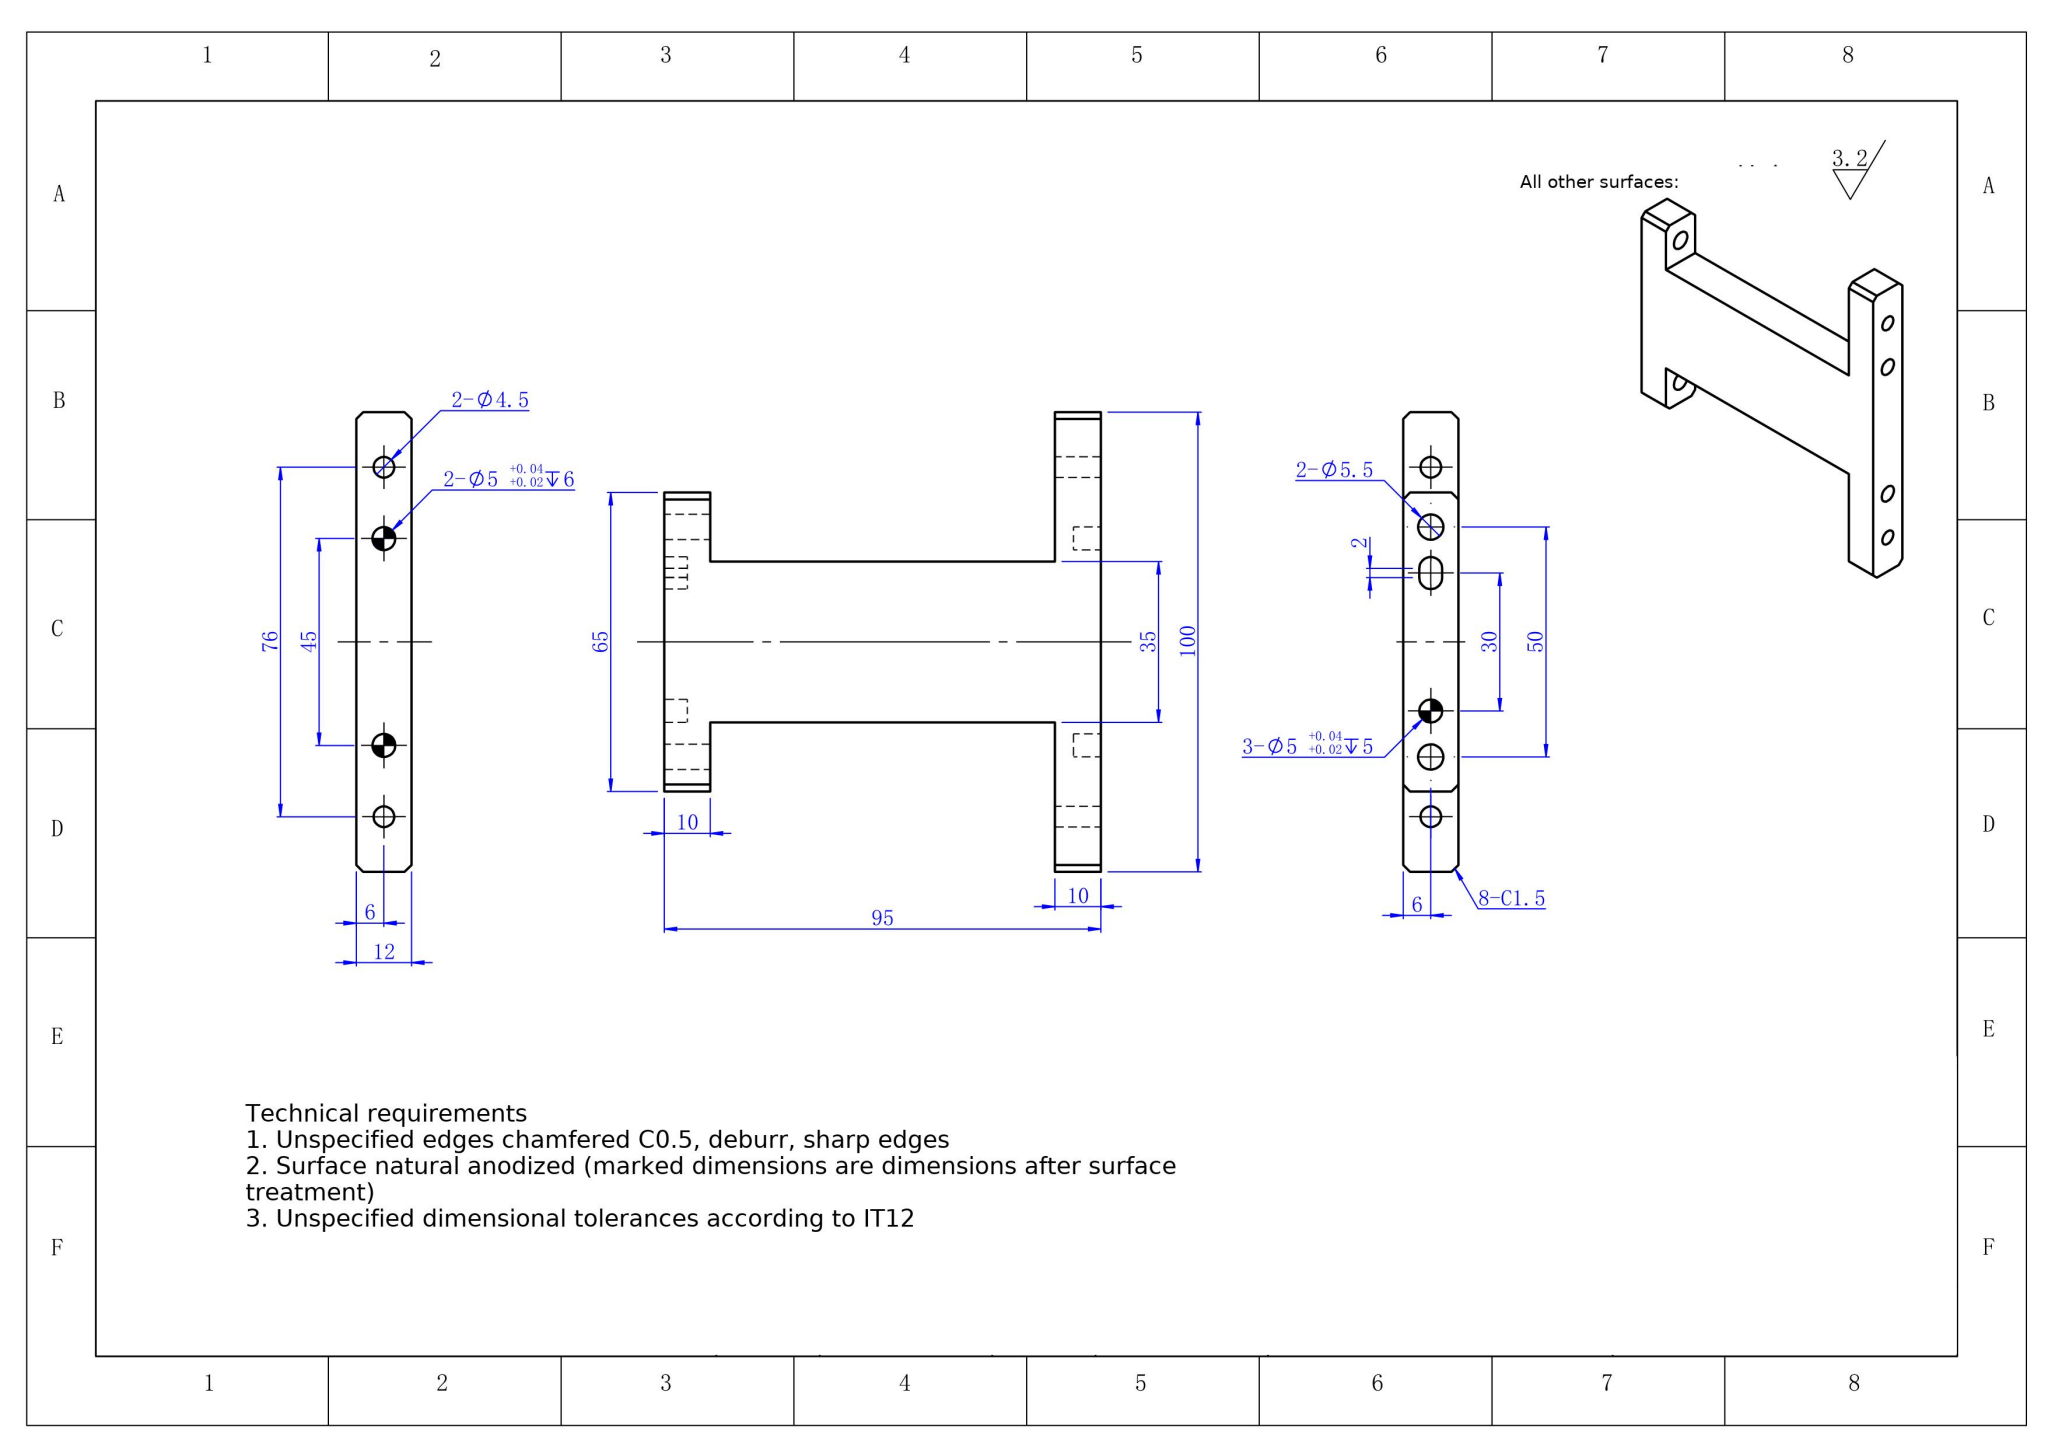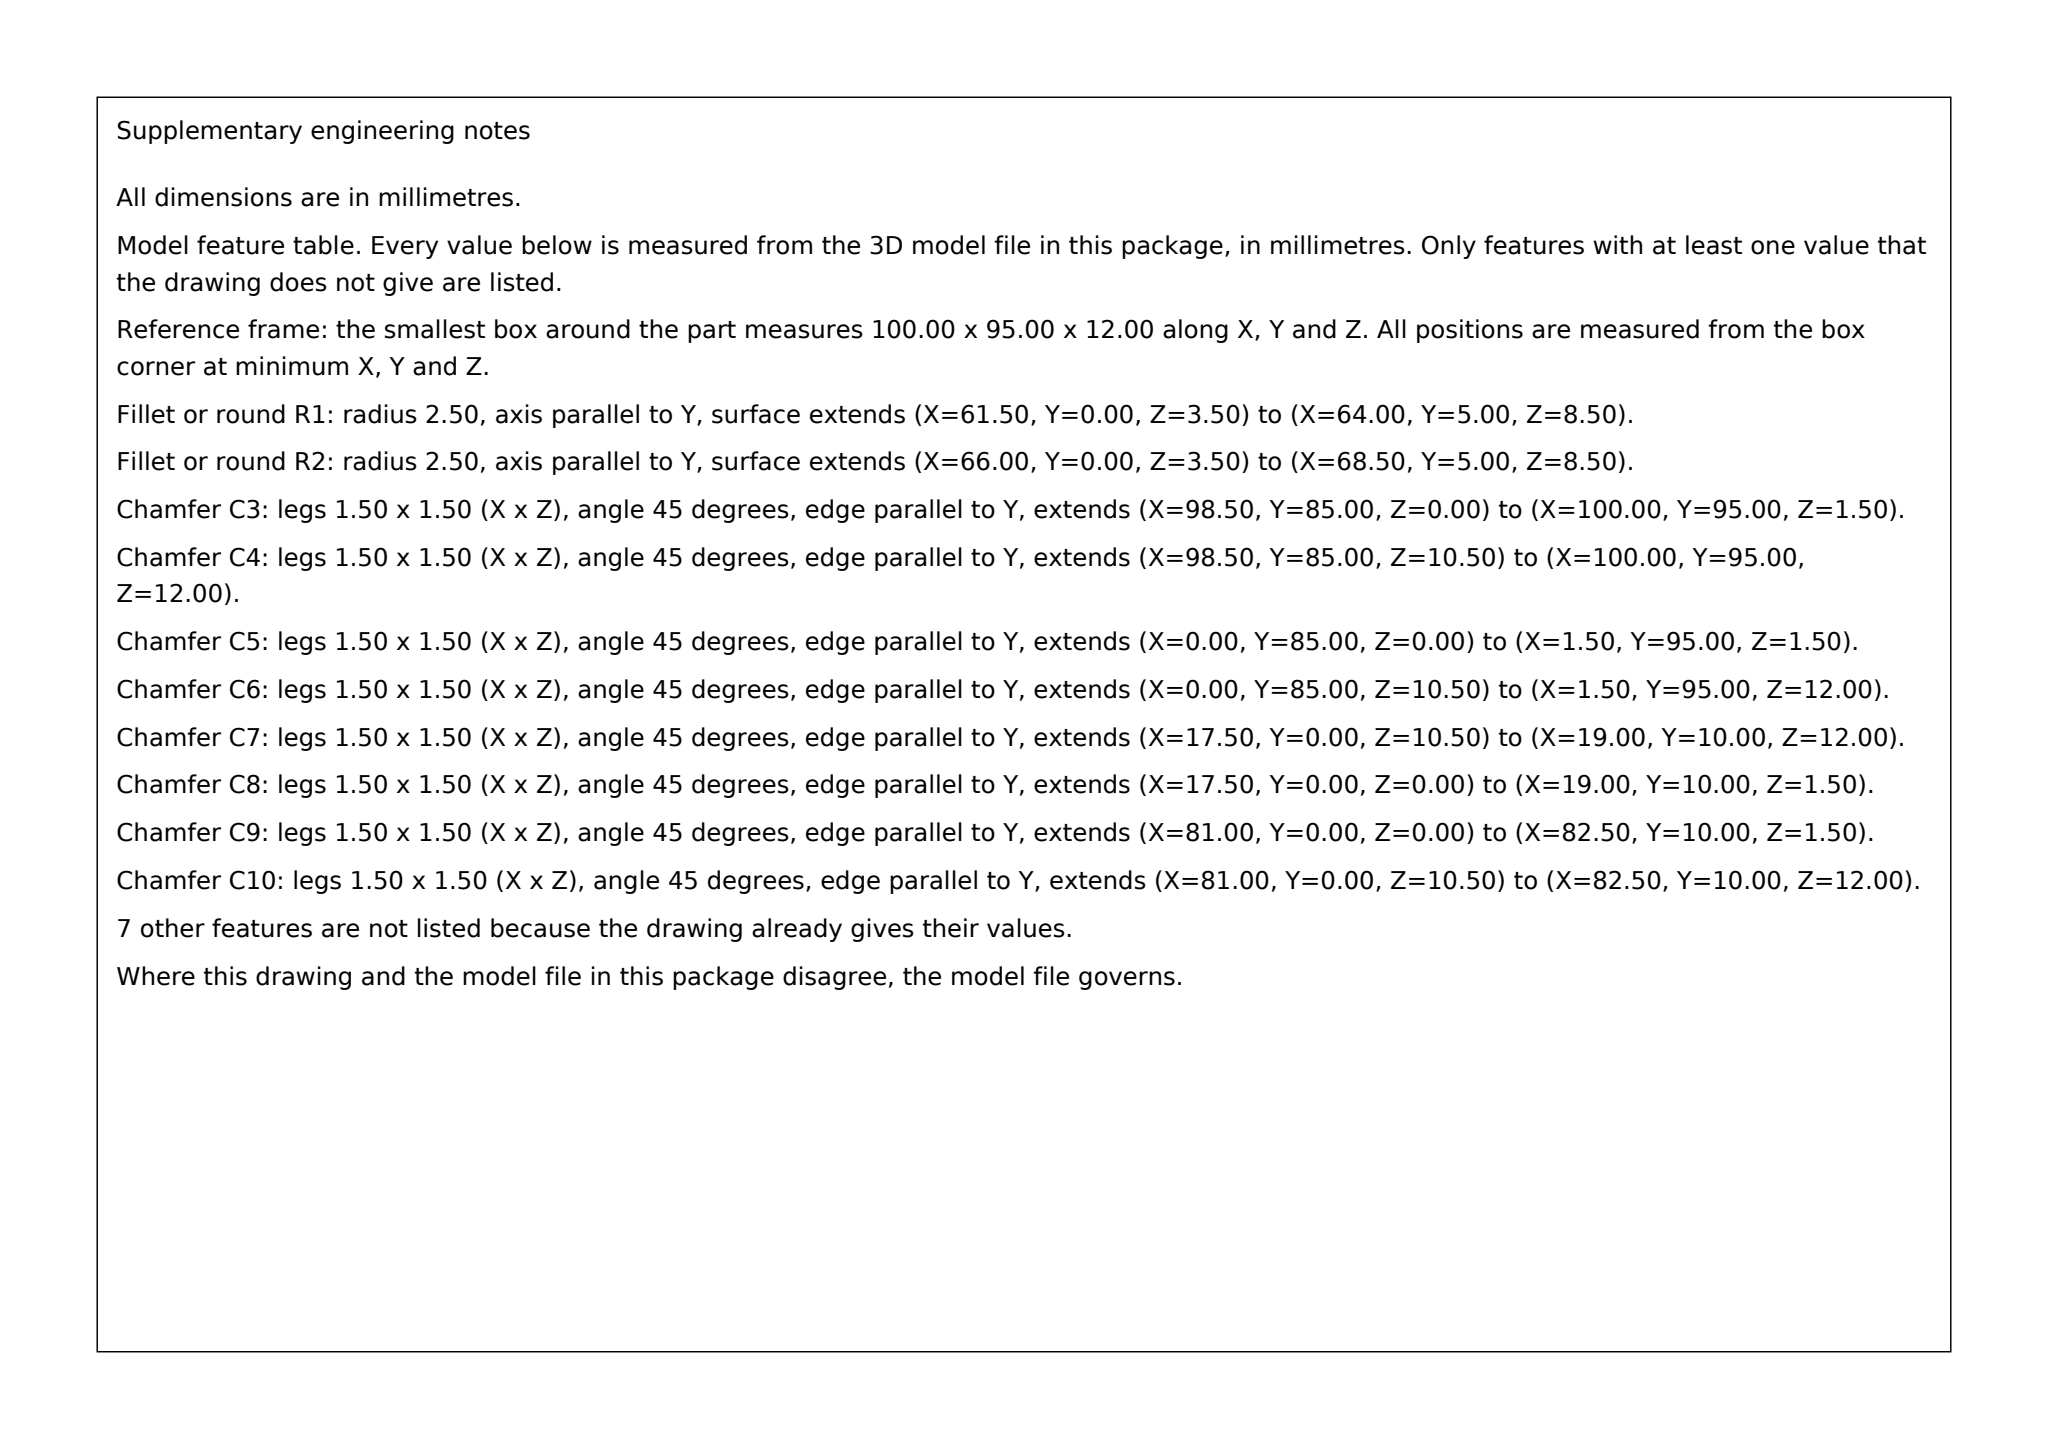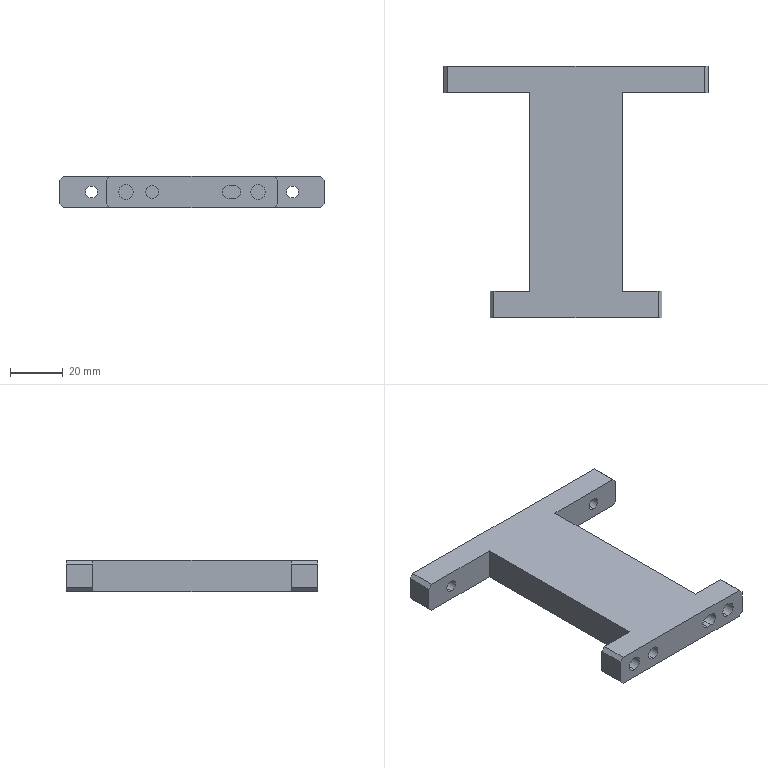Part | SolidWorks | mm | 1 solid | 44 faces | box 100 x 95 x 12 mm | volume 49935 mm3 | plane 28 | cylinder 16 | commonest cylinder face diameters 5 x8 4.5 x4 5.5 x4
build123d program:
from build123d import *

# Parameters (mm, degrees)
BOSS_EXTRUDE1_DEPTH        = 6
CUT_EXTRUDE1_REACH         = 109.522
SKETCH3_R                  = 2.75
F_4_5_4_5_DIAMETER_HOLE1_D = 4.5
SKETCH8_R                  = 2.5
CUT_EXTRUDE2_DEPTH         = 6
SKETCH9_R                  = 2.5
CUT_EXTRUDE3_DEPTH         = 5
CHAMFER1_SIZE              = 1.5


with BuildPart() as part:
    # Sketch2 → Boss-Extrude1 (new, symmetric)
    with BuildSketch(Plane.XY):
        Polygon((-32.5, 0), (32.5, 0), (32.5, 10), (17.5, 10), (17.5, 85), (50, 85), (50, 95), (-50, 95), (-50, 85), (-17.5, 85), (-17.5, 10), (-32.5, 10), align=None)
    extrude(amount=BOSS_EXTRUDE1_DEPTH, both=True)

    # Sketch3 → Cut-Extrude1 (cut, up to next)
    with BuildSketch(Plane.XZ, mode=Mode.PRIVATE) as cut_extrude1_sk1:
        with Locations(Location((-25, 0, 0), (0, 0, 270))):
            Circle(SKETCH3_R)
    cut_extrude1_tool1 = extrude(cut_extrude1_sk1.sketch, amount=-CUT_EXTRUDE1_REACH, mode=Mode.PRIVATE) & part.part
    # Sketch3 → Cut-Extrude1 (cut, up to next)
    with BuildSketch(Plane.XZ, mode=Mode.PRIVATE) as cut_extrude1_sk2:
        with Locations((25, 0)):
            Circle(SKETCH3_R)
    cut_extrude1_tool2 = extrude(cut_extrude1_sk2.sketch, amount=-CUT_EXTRUDE1_REACH, mode=Mode.PRIVATE) & part.part
    add(cut_extrude1_tool1.solids().sort_by_distance((-25, 0, 0))[0], mode=Mode.SUBTRACT)
    add(cut_extrude1_tool2.solids().sort_by_distance((25, 0, 0))[0], mode=Mode.SUBTRACT)

    # 4.5 _4.5_ Diameter Hole1 (through all)
    with Locations(Plane(origin=(0, 95, 0), x_dir=(1, 0, 0), z_dir=(0, 1, 0))):
        with Locations((-38, 0), (38, 0)):
            Hole(F_4_5_4_5_DIAMETER_HOLE1_D / 2)

    # Sketch8 → Cut-Extrude2 (cut)
    with BuildSketch(Plane(origin=(0, 95, 0), x_dir=(1, 0, 0), z_dir=(0, 1, 0))):
        with Locations(Location((-22.5, 0, 0), (0, 0, 270))):
            Circle(SKETCH8_R)
        with Locations(Location((22.5, 0, 0), (0, 0, 90))):
            Circle(SKETCH8_R)
    extrude(amount=-CUT_EXTRUDE2_DEPTH, mode=Mode.SUBTRACT)

    # Sketch9 → Cut-Extrude3 (cut)
    with BuildSketch(Plane.XZ):
        with Locations(Location((-15, 0, 0), (0, 0, 270))):
            Circle(SKETCH9_R)
        with BuildLine():
            Line((14, 2.5), (16, 2.5))
            ThreePointArc((16, 2.5), (18.5, 0), (16, -2.5))
            Line((16, -2.5), (14, -2.5))
            ThreePointArc((14, -2.5), (11.5, 0), (14, 2.5))
        make_face()
    extrude(amount=-CUT_EXTRUDE3_DEPTH, mode=Mode.SUBTRACT)

    # Chamfer1
    chamfer1_edges = [part.edges().sort_by_distance(p)[0] for p in [
        (32.5, 5, 6),
        (-50, 90, -6),
        (50, 90, -6),
        (32.5, 5, -6),
        (-32.5, 5, -6),
        (50, 90, 6),
        (-50, 90, 6),
        (-32.5, 5, 6),
    ]]
    chamfer(chamfer1_edges, length=CHAMFER1_SIZE)


solid = part.part